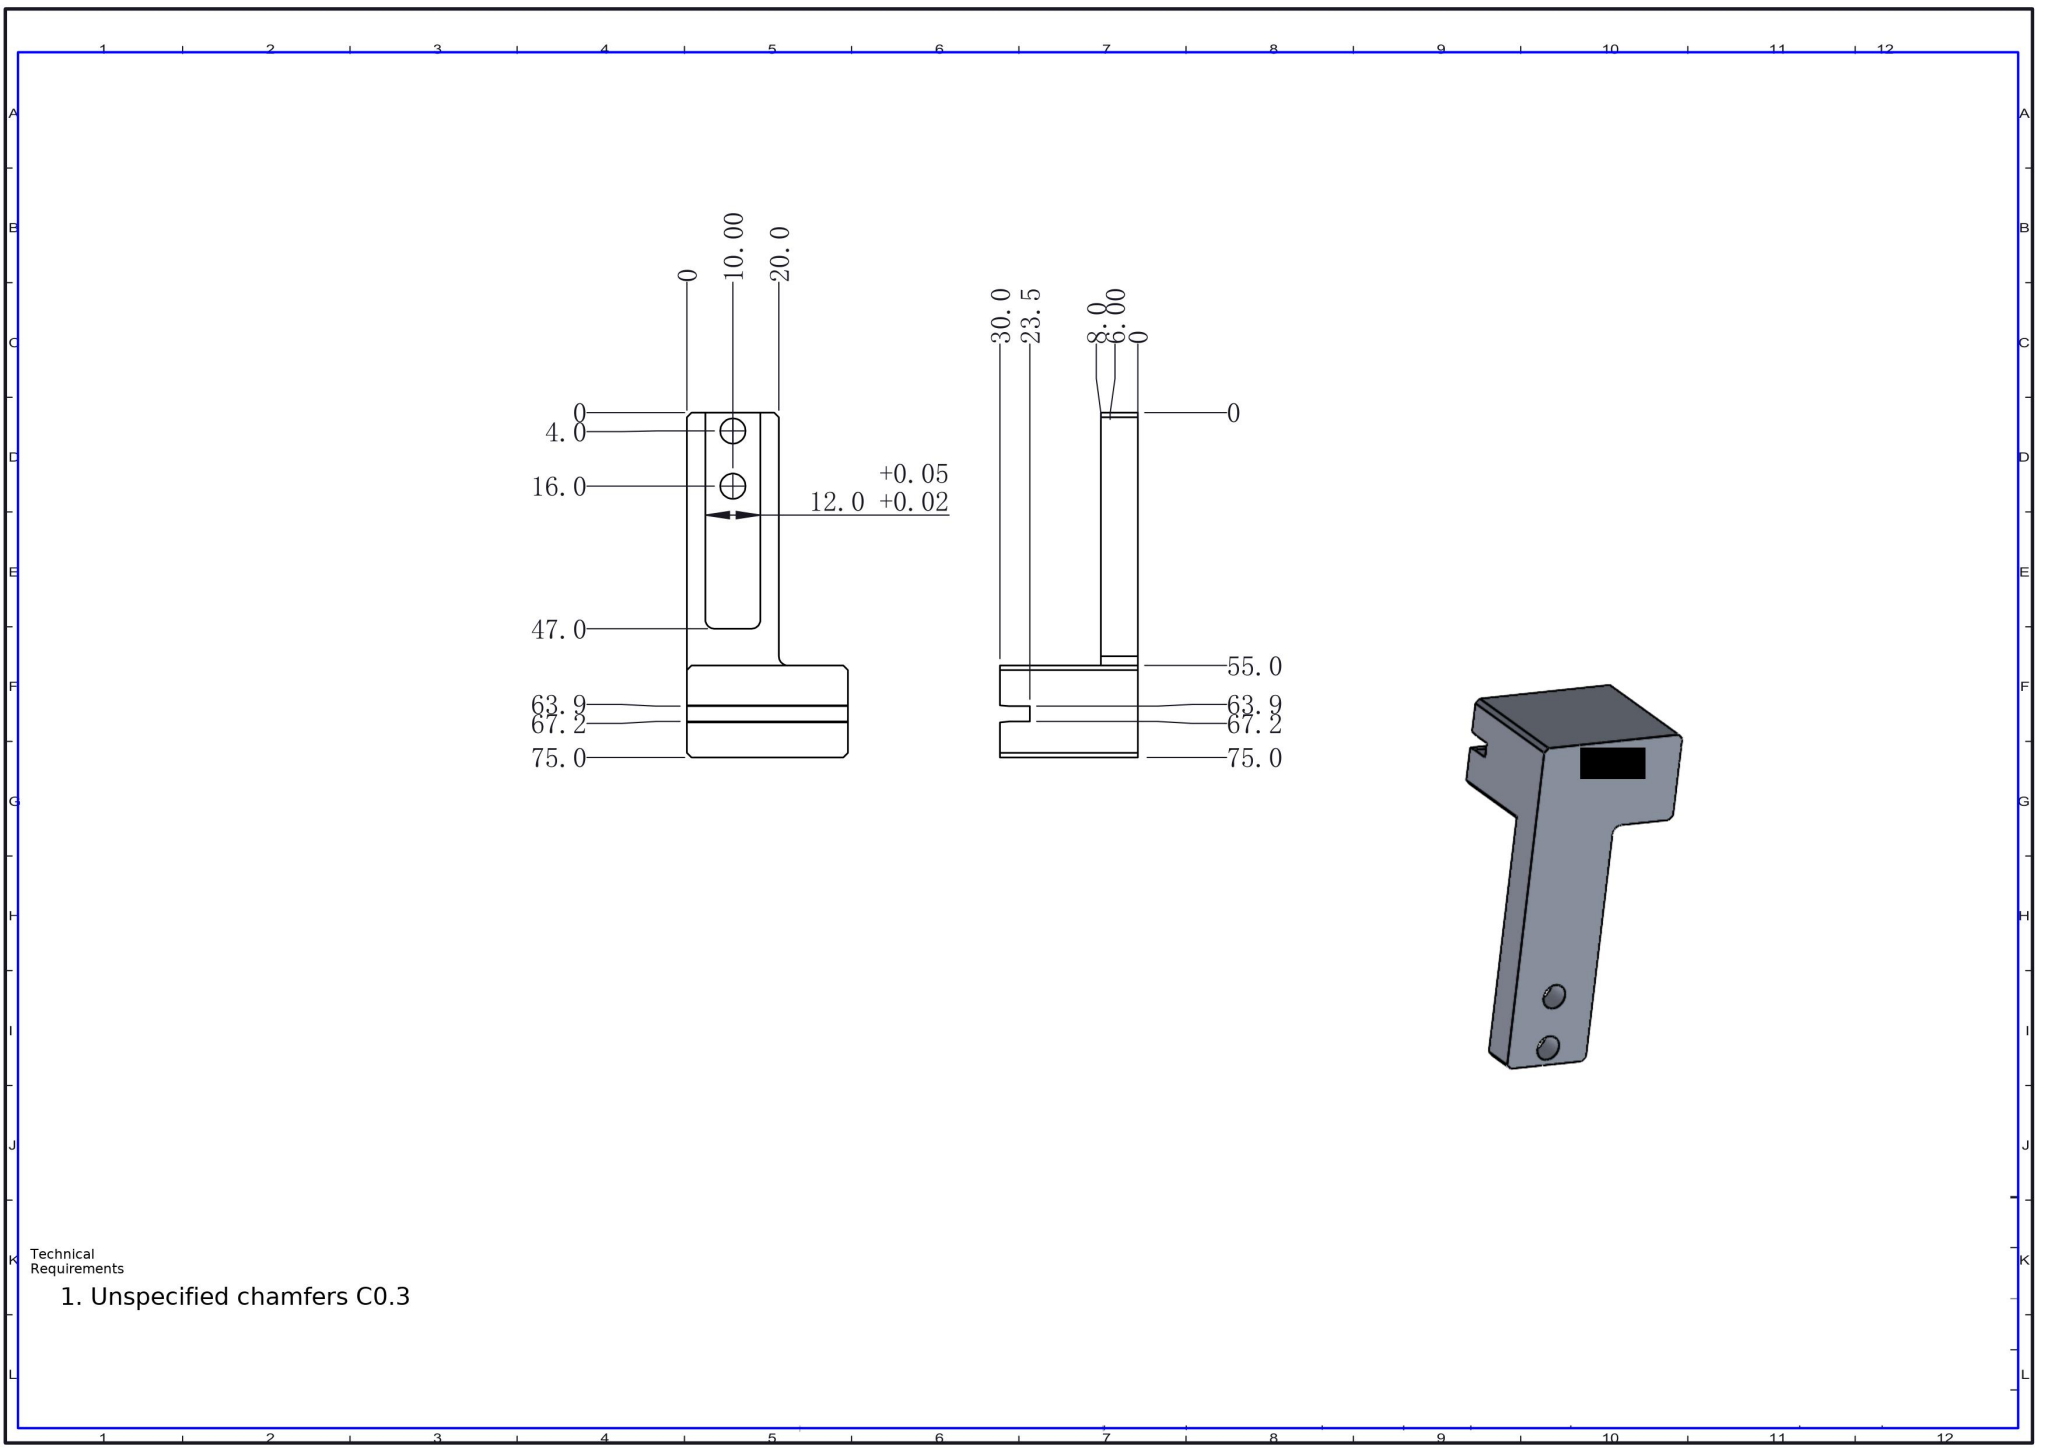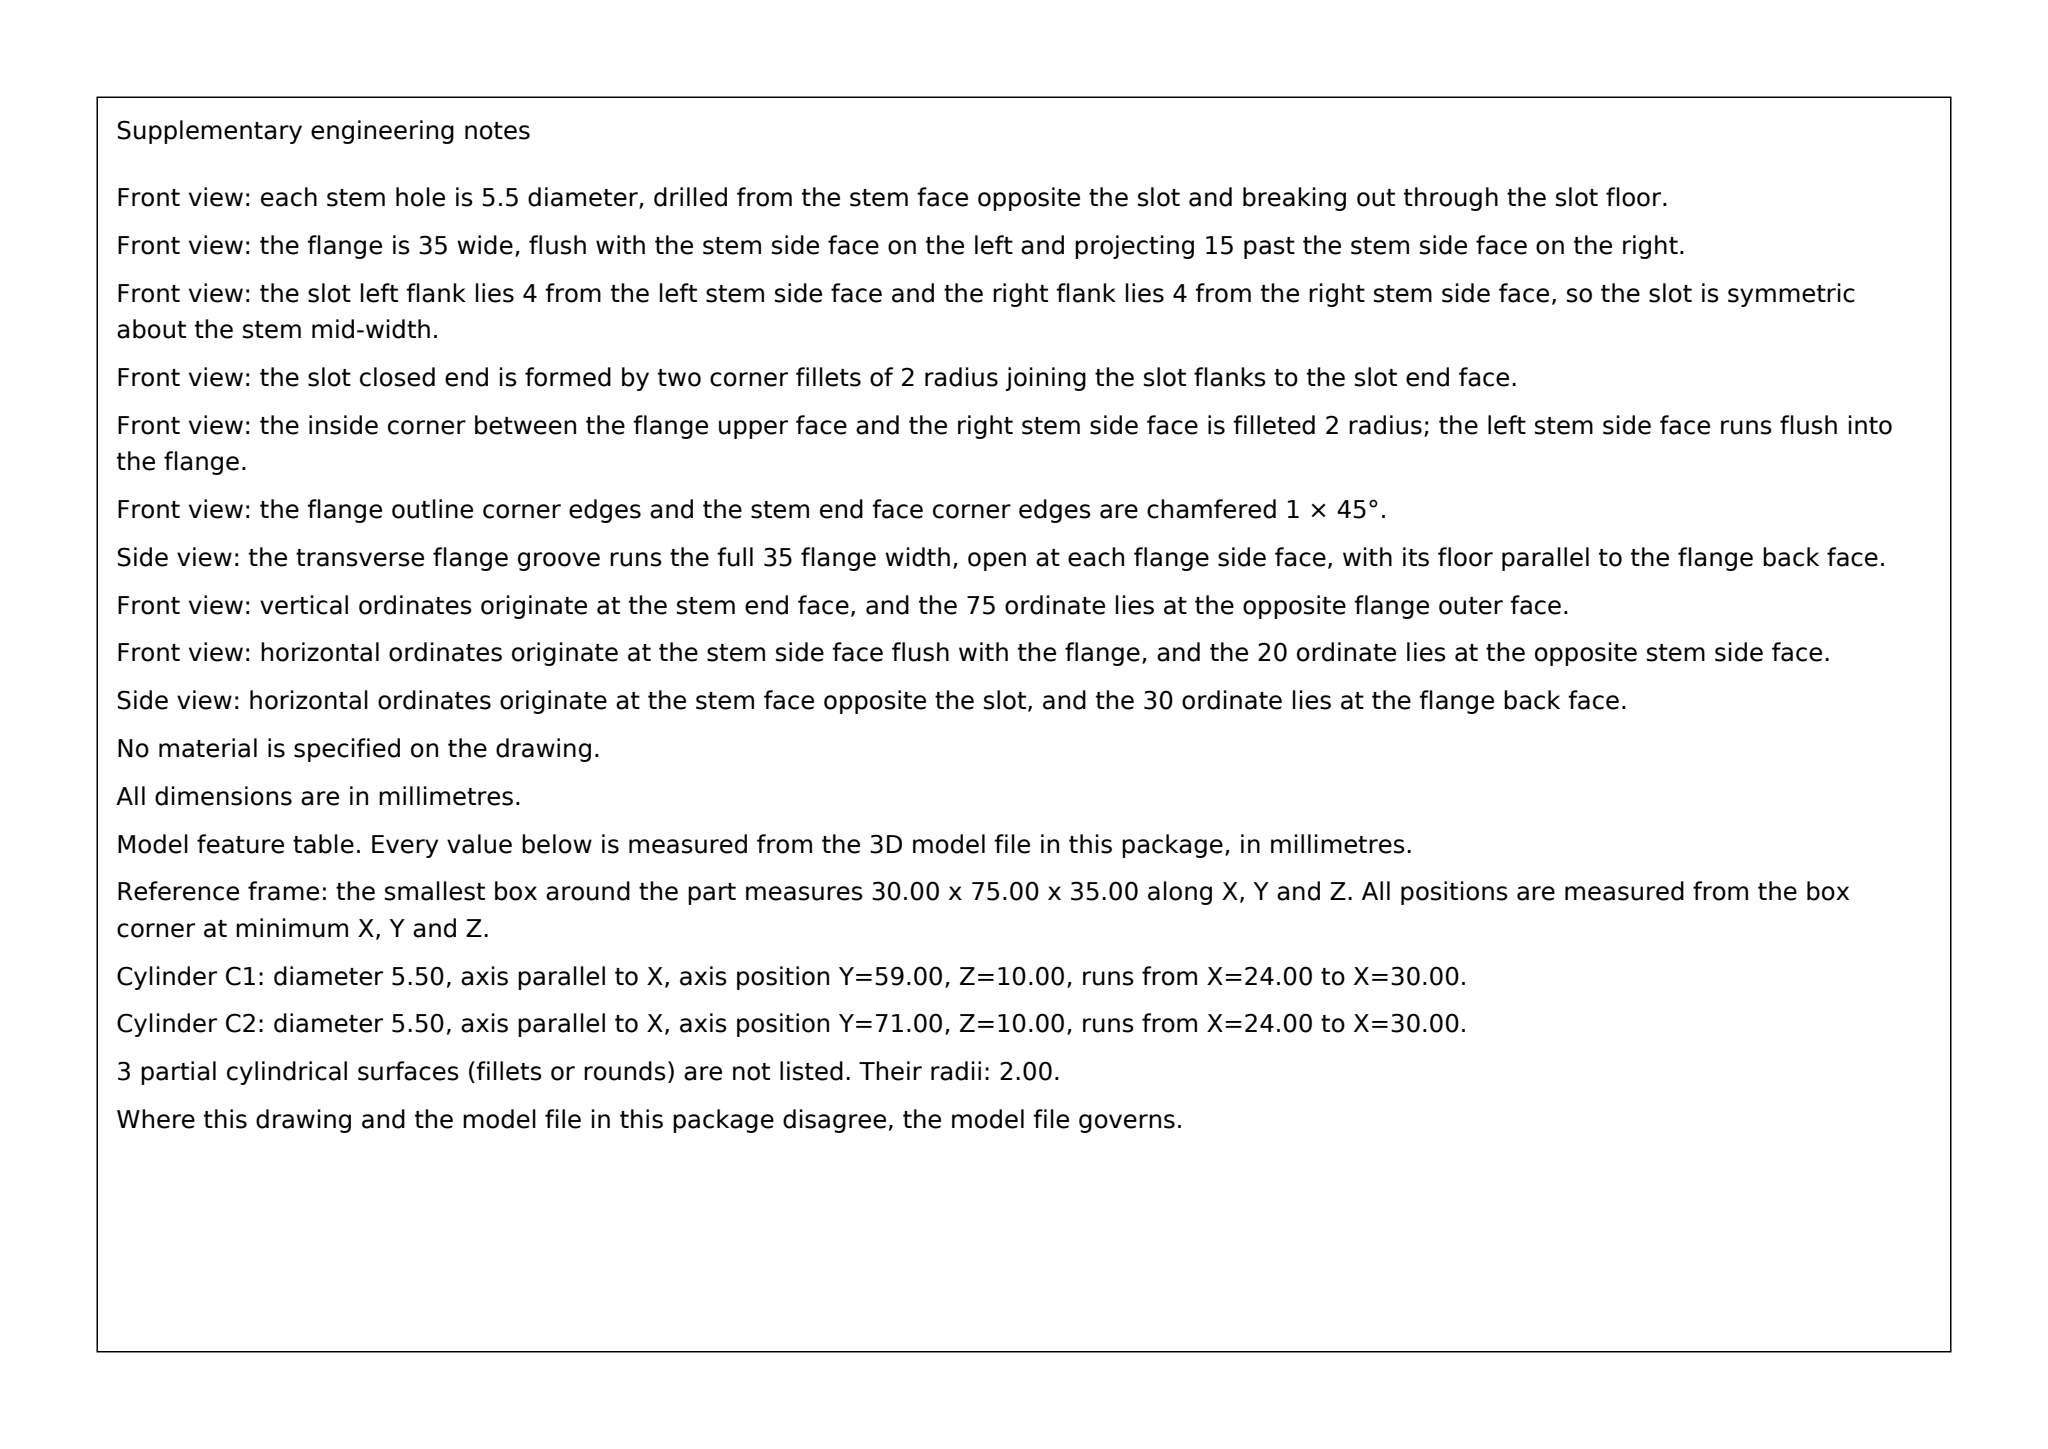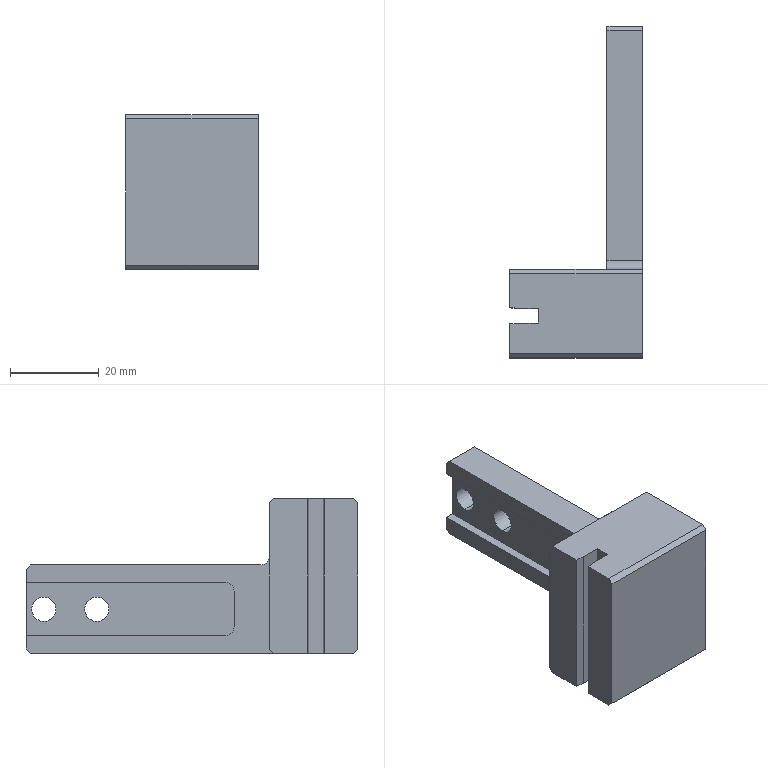Part | SolidWorks | mm | 1 solid | 216 faces | box 30 x 75 x 35 mm | volume 27567 mm3 | plane 124 | spline 85 | cylinder 7 | commonest cylinder face diameters 5.5 x4 4 x3
Drawing notes:
FRONT VIEW: 2X Ø5.5 DP 6, AT 4.0 & 16.0 BELOW TOP ORD | from the solid: cylinders [5.5,'x',[null,59.0,10.0],6.0] and [5.5,'x',[null,71.0,10.0],6.0]; bbox y=75 so 75-71=4.0, 75-59=16.0; axis at z=10.0 (10.00 ord); blind length 6.0
HEAD BLOCK 35.0 WIDE (0 TO 35.0 ORD); STEM 20.0 WIDE | from the solid: bbox_xyz z=35.0; axis_planes z=0.0 and z=35.0 bound head; z=20.0 plane = stem face matching 20.0 ordinate
TOP SLOT 2.0 WIDE: WALLS AT 6.0 AND 8.0 FROM THE 30.0 FACE (X=24.0 AND X=22.0 FROM MIN CORNER) | from the solid: axis_planes x=22.0 and x=24.0 (bbox x=30.0)
TOP SLOT ENDS Ø4.0 FULL RADIUS, AXES PARALLEL TO X AT Y=30.0, Z=6.0 AND Z=14.0 FROM MIN CORNER; SLOT DEPTH 2.0 | from the solid: cylinders [4.0,"x",[null,30.0,6.0],2.0] and [4.0,"x",[null,30.0,14.0],2.0]
ENGRAVE PART MARKING 'tcb_az07b' 0.2 DEEP ON THE X=30.0 FACE (ENGRAVED FLOOR AT X=29.8) | from the solid: axis_planes x=30.0 (outer face) and x=29.8 (9 recessed faces), 0.2 offset
FILLET R2.0 (Ø4.0 BLEND) AT STEM-TO-HEAD-BLOCK JUNCTION; AXIS PARALLEL TO X AT Y=22.0, Z=22.0 FROM MIN CORNER, 8.0 LONG ACROSS STEM THICKNESS | from the solid: cylinders[dia,axis,pos_other_axes,length]: [4.0,"x",[null,22.0,22.0],8.0,1]